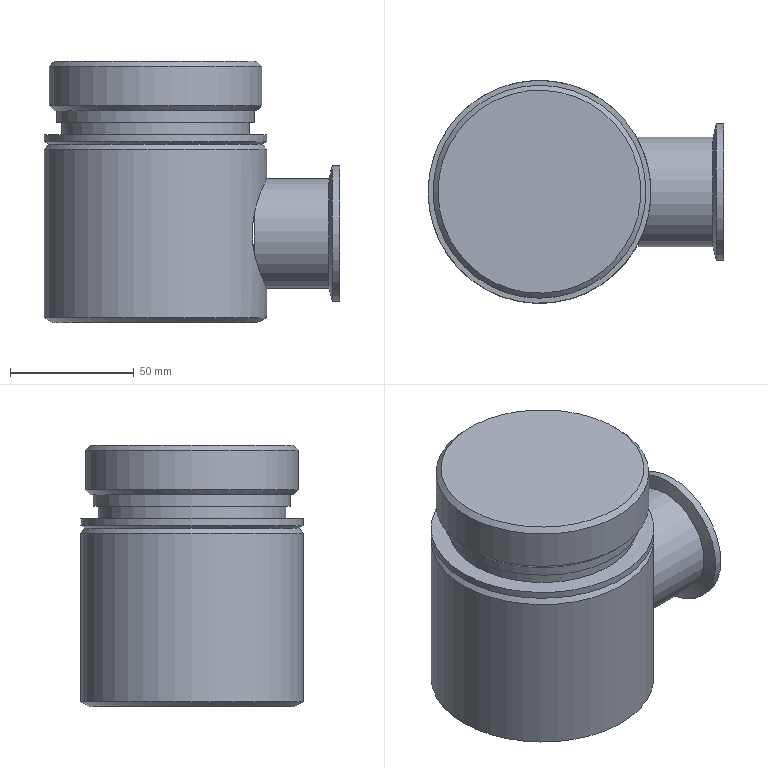Assembly | NX | mm | 5 component files | 5 solids | 47 faces | box 119.5 x 90 x 105.55 mm | volume 263374 mm3 | plane 20 | cylinder 19 | cone 8 | commonest cylinder face diameters 80 x4 74 x2 44.5 x2 90 x2 86 x1 82 x1 20 x1 55 x1
Bill of materials:
CH3404.19.3-4 | 1 |  | Flanged cylindrical sleeve: a hollow straight cylinder with a through bore and a thin, larger-diameter flange at one end; the flange has a tapered (conical) transition on the side facing the body.
CH3404.19.3-6 | 1 |  | Flanged plug with a tapered shank: a thin circular flange with chamfered edges on top of a conical body that narrows away from the flange, with a small central hole in the flange face.
CH3404.19.3-3 | 1 |  | Thin-walled cylindrical tube with chamfered end edges and a single round radial hole through the wall.
CH3404.19.3-1 | 1 |  | Solid short circular disc (puck) with chamfered edges on both faces.
CH3404.19.3-2 | 1 |  | Stepped ring with a through bore: a short cylindrical body with a reduced-diameter neck, a thin projecting flange with a chamfered edge, and a short cylindrical section below the flange; the bore appears stepped (counterbored) from the top end.
Mates:
1. touch align | CH3404_19_3-3 1 | assembly datumplane
2. touch align | CH3404_19_3-3 1 face | assembly datumaxis
3. touch align | CH3404_19_3-2 1 face | CH3404_19_3-3 1 face
4. touch align | CH3404_19_3-2 1 | assembly datumplane
5. touch align | CH3404_19_3-2 1 face | assembly datumaxis
6. touch align | CH3404_19_3-6 1 | assembly datumplane
7. touch align | CH3404_19_3-6 1 face | assembly datumaxis
8. touch align | CH3404_19_3-1 1 face | CH3404_19_3-6 1 face
9. touch align | CH3404_19_3-1 1 datumplane | assembly datumplane
10. touch align | CH3404_19_3-1 1 face | assembly datumaxis
11. touch align | CH3404_19_3-4 1 face | assembly datumplane
12. touch align | CH3404_19_3-4 1 face | CH3404_19_3-3 1 face